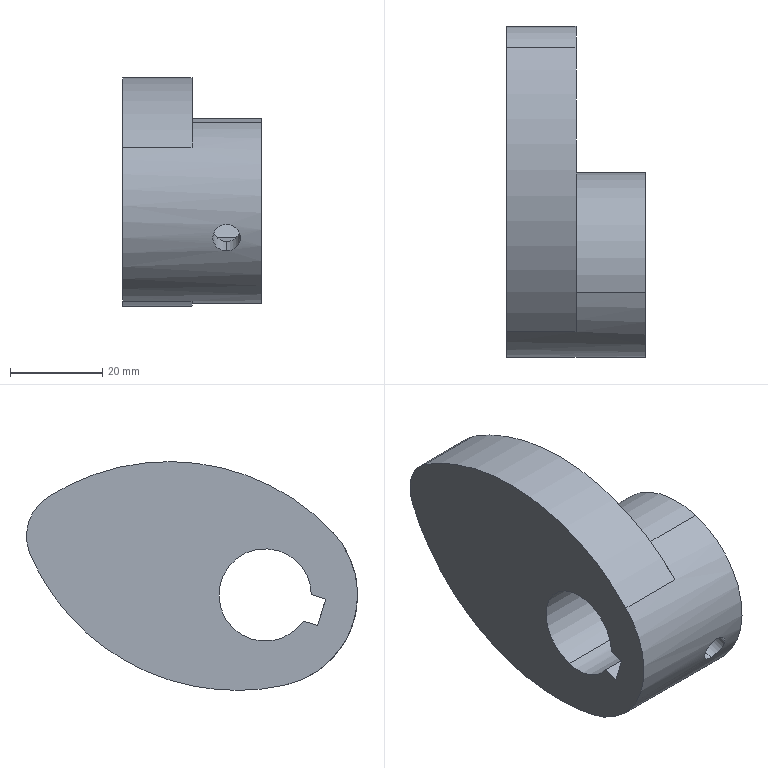Component | SolidWorks | ZL-11-11Cam2-1 | 1 solid | 20 faces | box 30 x 71.7 x 49.54 mm | volume 48547 mm3 | cylinder 13 | plane 7 | commonest cylinder face diameters 6 x4 20 x4 97.465 x3 40 x2
STEP:
#1=COLOUR_RGB('',0.7922,0.8196,0.9333);
#2=FILL_AREA_STYLE_COLOUR('',#1);
#3=FILL_AREA_STYLE('',(#2));
#4=SURFACE_STYLE_FILL_AREA(#3);
#5=SURFACE_SIDE_STYLE('',(#4));
#6=SURFACE_STYLE_USAGE(.BOTH.,#5);
#7=PRESENTATION_STYLE_ASSIGNMENT((#6));
#8=CARTESIAN_POINT('',(-2.2,4.601,-0.3247));
#9=VERTEX_POINT('',#8);
#10=CARTESIAN_POINT('',(-2.082,4.494,-0.3765));
#11=VERTEX_POINT('',#10);
#12=CARTESIAN_POINT('',(-2.2,4.601,-0.3247));
#13=CARTESIAN_POINT('',(-2.192,4.601,-0.3247));
#14=CARTESIAN_POINT('',(-2.184,4.601,-0.3251));
#15=CARTESIAN_POINT('',(-2.169,4.598,-0.3269));
#16=CARTESIAN_POINT('',(-2.161,4.596,-0.3282));
#17=CARTESIAN_POINT('',(-2.147,4.591,-0.3316));
#18=CARTESIAN_POINT('',(-2.14,4.588,-0.3337));
#19=CARTESIAN_POINT('',(-2.128,4.58,-0.3383));
#20=CARTESIAN_POINT('',(-2.122,4.576,-0.3408));
#21=CARTESIAN_POINT('',(-2.111,4.566,-0.3463));
#22=CARTESIAN_POINT('',(-2.106,4.561,-0.3491));
#23=CARTESIAN_POINT('',(-2.097,4.549,-0.3549));
#24=CARTESIAN_POINT('',(-2.094,4.543,-0.3579));
#25=CARTESIAN_POINT('',(-2.088,4.53,-0.3637));
#26=CARTESIAN_POINT('',(-2.085,4.523,-0.3664));
#27=CARTESIAN_POINT('',(-2.082,4.509,-0.3717));
#28=CARTESIAN_POINT('',(-2.082,4.501,-0.3742));
#29=CARTESIAN_POINT('',(-2.082,4.494,-0.3765));
#30=B_SPLINE_CURVE_WITH_KNOTS('',3,(#12,#13,#14,#15,#16,#17,#18,#19,#20,#21,#22,#23,#24,#25,#26,#27,#28,#29),.UNSPECIFIED.,.F.,.F.,(4,2,2,2,2,2,2,2,4),(0.009434,0.01002,0.01061,0.0112,0.01179,0.01238,0.01297,0.01356,0.01415),.UNSPECIFIED.);
#31=EDGE_CURVE('',#9,#11,#30,.T.);
#32=ORIENTED_EDGE('',*,*,#31,.F.);
#33=CARTESIAN_POINT('',(-2.2,4.719,-0.71));
#34=VERTEX_POINT('',#33);
#35=CARTESIAN_POINT('',(-2.2,4.722,-0.7185));
#36=DIRECTION('',(-0.,0.2922,-0.9564));
#37=VECTOR('',#36,39.37);
#38=LINE('',#35,#37);
#39=EDGE_CURVE('',#9,#34,#38,.T.);
#40=ORIENTED_EDGE('',*,*,#39,.T.);
#41=CARTESIAN_POINT('',(-2.082,4.609,-0.753));
#42=VERTEX_POINT('',#41);
#43=CARTESIAN_POINT('',(-2.082,4.609,-0.753));
#44=CARTESIAN_POINT('',(-2.082,4.616,-0.7508));
#45=CARTESIAN_POINT('',(-2.082,4.623,-0.7484));
#46=CARTESIAN_POINT('',(-2.085,4.638,-0.7435));
#47=CARTESIAN_POINT('',(-2.088,4.645,-0.7411));
#48=CARTESIAN_POINT('',(-2.094,4.658,-0.7361));
#49=CARTESIAN_POINT('',(-2.097,4.665,-0.7336));
#50=CARTESIAN_POINT('',(-2.106,4.677,-0.7288));
#51=CARTESIAN_POINT('',(-2.111,4.682,-0.7265));
#52=CARTESIAN_POINT('',(-2.122,4.692,-0.7223));
#53=CARTESIAN_POINT('',(-2.128,4.697,-0.7202));
#54=CARTESIAN_POINT('',(-2.14,4.705,-0.7167));
#55=CARTESIAN_POINT('',(-2.147,4.708,-0.7152));
#56=CARTESIAN_POINT('',(-2.162,4.714,-0.7126));
#57=CARTESIAN_POINT('',(-2.169,4.716,-0.7117));
#58=CARTESIAN_POINT('',(-2.184,4.718,-0.7103));
#59=CARTESIAN_POINT('',(-2.192,4.719,-0.71));
#60=CARTESIAN_POINT('',(-2.2,4.719,-0.71));
#61=B_SPLINE_CURVE_WITH_KNOTS('',3,(#43,#44,#45,#46,#47,#48,#49,#50,#51,#52,#53,#54,#55,#56,#57,#58,#59,#60),.UNSPECIFIED.,.F.,.F.,(4,2,2,2,2,2,2,2,4),(0.009393,0.00998,0.01057,0.01115,0.01174,0.01233,0.01292,0.0135,0.01409),.UNSPECIFIED.);
#62=EDGE_CURVE('',#42,#34,#61,.T.);
#63=ORIENTED_EDGE('',*,*,#62,.F.);
#64=CARTESIAN_POINT('',(-2.2,4.493,-0.779));
#65=VERTEX_POINT('',#64);
#66=CARTESIAN_POINT('',(-2.2,4.493,-0.779));
#67=CARTESIAN_POINT('',(-2.192,4.493,-0.779));
#68=CARTESIAN_POINT('',(-2.184,4.494,-0.7789));
#69=CARTESIAN_POINT('',(-2.169,4.497,-0.7785));
#70=CARTESIAN_POINT('',(-2.162,4.499,-0.7781));
#71=CARTESIAN_POINT('',(-2.147,4.505,-0.7772));
#72=CARTESIAN_POINT('',(-2.14,4.509,-0.7766));
#73=CARTESIAN_POINT('',(-2.128,4.517,-0.7751));
#74=CARTESIAN_POINT('',(-2.122,4.522,-0.7742));
#75=CARTESIAN_POINT('',(-2.111,4.533,-0.7721));
#76=CARTESIAN_POINT('',(-2.106,4.539,-0.771));
#77=CARTESIAN_POINT('',(-2.097,4.551,-0.7682));
#78=CARTESIAN_POINT('',(-2.094,4.558,-0.7667));
#79=CARTESIAN_POINT('',(-2.088,4.572,-0.7633));
#80=CARTESIAN_POINT('',(-2.085,4.579,-0.7615));
#81=CARTESIAN_POINT('',(-2.082,4.594,-0.7575));
#82=CARTESIAN_POINT('',(-2.082,4.601,-0.7553));
#83=CARTESIAN_POINT('',(-2.082,4.609,-0.753));
#84=B_SPLINE_CURVE_WITH_KNOTS('',3,(#66,#67,#68,#69,#70,#71,#72,#73,#74,#75,#76,#77,#78,#79,#80,#81,#82,#83),.UNSPECIFIED.,.F.,.F.,(4,2,2,2,2,2,2,2,4),(0.004697,0.005284,0.005871,0.006458,0.007045,0.007632,0.008219,0.008806,0.009393),.UNSPECIFIED.);
#85=EDGE_CURVE('',#65,#42,#84,.T.);
#86=ORIENTED_EDGE('',*,*,#85,.F.);
#87=CARTESIAN_POINT('',(-2.2,4.376,-0.3937));
#88=VERTEX_POINT('',#87);
#89=CARTESIAN_POINT('',(-2.2,4.496,-0.7876));
#90=DIRECTION('',(-0.,0.2922,-0.9564));
#91=VECTOR('',#90,39.37);
#92=LINE('',#89,#91);
#93=EDGE_CURVE('',#88,#65,#92,.T.);
#94=ORIENTED_EDGE('',*,*,#93,.F.);
#95=CARTESIAN_POINT('',(-2.082,4.494,-0.3765));
#96=CARTESIAN_POINT('',(-2.082,4.486,-0.3788));
#97=CARTESIAN_POINT('',(-2.082,4.479,-0.3808));
#98=CARTESIAN_POINT('',(-2.085,4.464,-0.3844));
#99=CARTESIAN_POINT('',(-2.088,4.457,-0.386));
#100=CARTESIAN_POINT('',(-2.097,4.436,-0.3898));
#101=CARTESIAN_POINT('',(-2.105,4.422,-0.3914));
#102=CARTESIAN_POINT('',(-2.122,4.406,-0.3928));
#103=CARTESIAN_POINT('',(-2.128,4.401,-0.3931));
#104=CARTESIAN_POINT('',(-2.14,4.392,-0.3935));
#105=CARTESIAN_POINT('',(-2.147,4.388,-0.3936));
#106=CARTESIAN_POINT('',(-2.161,4.382,-0.3937));
#107=CARTESIAN_POINT('',(-2.169,4.379,-0.3937));
#108=CARTESIAN_POINT('',(-2.184,4.376,-0.3937));
#109=CARTESIAN_POINT('',(-2.192,4.376,-0.3937));
#110=CARTESIAN_POINT('',(-2.2,4.376,-0.3937));
#111=B_SPLINE_CURVE_WITH_KNOTS('',3,(#95,#96,#97,#98,#99,#100,#101,#102,#103,#104,#105,#106,#107,#108,#109,#110),.UNSPECIFIED.,.F.,.F.,(4,2,2,2,2,2,2,4),(0.01415,0.01474,0.01533,0.01651,0.0171,0.01769,0.01828,0.01887),.UNSPECIFIED.);
#112=EDGE_CURVE('',#11,#88,#111,.T.);
#113=ORIENTED_EDGE('',*,*,#112,.F.);
#114=EDGE_LOOP('',(#32,#40,#63,#86,#94,#113));
#115=FACE_OUTER_BOUND('',#114,.T.);
#116=CARTESIAN_POINT('',(-2.2,4.609,-0.753));
#117=DIRECTION('',(-0.,0.2922,-0.9564));
#118=DIRECTION('',(0.,-0.9564,-0.2922));
#119=AXIS2_PLACEMENT_3D('',#116,#117,#118);
#120=CYLINDRICAL_SURFACE('',#119,0.1181);
#121=ADVANCED_FACE('',(#115),#120,.F.);
#122=CARTESIAN_POINT('',(-2.2,3.931,-0.2602));
#123=VERTEX_POINT('',#122);
#124=CARTESIAN_POINT('',(-2.2,3.862,-0.03428));
#125=VERTEX_POINT('',#124);
#126=CARTESIAN_POINT('',(-2.2,3.897,-0.1472));
#127=DIRECTION('',(0.,-0.9564,-0.2922));
#128=DIRECTION('',(0.,-0.2922,0.9564));
#129=AXIS2_PLACEMENT_3D('',#126,#127,#128);
#130=CIRCLE('',#129,0.1181);
#131=EDGE_CURVE('',#123,#125,#130,.T.);
#132=ORIENTED_EDGE('',*,*,#131,.F.);
#133=CARTESIAN_POINT('',(-2.2,3.669,-0.3404));
#134=VERTEX_POINT('',#133);
#135=CARTESIAN_POINT('',(-2.2,3.66,-0.343));
#136=DIRECTION('',(0.,-0.9564,-0.2922));
#137=VECTOR('',#136,39.37);
#138=LINE('',#135,#137);
#139=EDGE_CURVE('',#123,#134,#138,.T.);
#140=ORIENTED_EDGE('',*,*,#139,.T.);
#141=CARTESIAN_POINT('',(-2.2,3.6,-0.1145));
#142=VERTEX_POINT('',#141);
#143=CARTESIAN_POINT('',(-2.2,3.6,-0.1145));
#144=CARTESIAN_POINT('',(-2.192,3.6,-0.1145));
#145=CARTESIAN_POINT('',(-2.184,3.6,-0.1153));
#146=CARTESIAN_POINT('',(-2.169,3.6,-0.1183));
#147=CARTESIAN_POINT('',(-2.162,3.601,-0.1206));
#148=CARTESIAN_POINT('',(-2.147,3.602,-0.1265));
#149=CARTESIAN_POINT('',(-2.141,3.602,-0.1301));
#150=CARTESIAN_POINT('',(-2.128,3.604,-0.1386));
#151=CARTESIAN_POINT('',(-2.122,3.604,-0.1435));
#152=CARTESIAN_POINT('',(-2.111,3.607,-0.1543));
#153=CARTESIAN_POINT('',(-2.106,3.608,-0.1601));
#154=CARTESIAN_POINT('',(-2.097,3.61,-0.1728));
#155=CARTESIAN_POINT('',(-2.094,3.612,-0.1795));
#156=CARTESIAN_POINT('',(-2.088,3.615,-0.1933));
#157=CARTESIAN_POINT('',(-2.085,3.617,-0.2006));
#158=CARTESIAN_POINT('',(-2.082,3.621,-0.2153));
#159=CARTESIAN_POINT('',(-2.082,3.623,-0.2226));
#160=CARTESIAN_POINT('',(-2.082,3.628,-0.2374));
#161=CARTESIAN_POINT('',(-2.082,3.63,-0.2449));
#162=CARTESIAN_POINT('',(-2.085,3.635,-0.2592));
#163=CARTESIAN_POINT('',(-2.088,3.638,-0.2662));
#164=CARTESIAN_POINT('',(-2.094,3.643,-0.2796));
#165=CARTESIAN_POINT('',(-2.097,3.645,-0.2861));
#166=CARTESIAN_POINT('',(-2.106,3.65,-0.298));
#167=CARTESIAN_POINT('',(-2.111,3.652,-0.3035));
#168=CARTESIAN_POINT('',(-2.122,3.657,-0.3137));
#169=CARTESIAN_POINT('',(-2.128,3.658,-0.3182));
#170=CARTESIAN_POINT('',(-2.14,3.662,-0.3261));
#171=CARTESIAN_POINT('',(-2.147,3.664,-0.3295));
#172=CARTESIAN_POINT('',(-2.162,3.666,-0.3349));
#173=CARTESIAN_POINT('',(-2.169,3.667,-0.337));
#174=CARTESIAN_POINT('',(-2.184,3.668,-0.3397));
#175=CARTESIAN_POINT('',(-2.192,3.669,-0.3404));
#176=CARTESIAN_POINT('',(-2.2,3.669,-0.3404));
#177=B_SPLINE_CURVE_WITH_KNOTS('',3,(#143,#144,#145,#146,#147,#148,#149,#150,#151,#152,#153,#154,#155,#156,#157,#158,#159,#160,#161,#162,#163,#164,#165,#166,#167,#168,#169,#170,#171,#172,#173,#174,#175,#176),.UNSPECIFIED.,.F.,.F.,(4,2,2,2,2,2,2,2,2,2,2,2,2,2,2,2,4),(0.,0.000587,0.001174,0.001761,0.002348,0.002935,0.003522,0.004109,0.004696,0.005283,0.00587,0.006457,0.007044,0.007631,0.008219,0.008806,0.009393),.UNSPECIFIED.);
#178=EDGE_CURVE('',#142,#134,#177,.T.);
#179=ORIENTED_EDGE('',*,*,#178,.F.);
#180=CARTESIAN_POINT('',(-2.2,3.591,-0.1171));
#181=DIRECTION('',(0.,-0.9564,-0.2922));
#182=VECTOR('',#181,39.37);
#183=LINE('',#180,#182);
#184=EDGE_CURVE('',#125,#142,#183,.T.);
#185=ORIENTED_EDGE('',*,*,#184,.F.);
#186=EDGE_LOOP('',(#132,#140,#179,#185));
#187=FACE_OUTER_BOUND('',#186,.T.);
#188=CARTESIAN_POINT('',(-2.2,3.626,-0.2301));
#189=DIRECTION('',(0.,-0.9564,-0.2922));
#190=DIRECTION('',(0.,-0.2922,0.9564));
#191=AXIS2_PLACEMENT_3D('',#188,#189,#190);
#192=CYLINDRICAL_SURFACE('',#191,0.1181);
#193=ADVANCED_FACE('',(#187),#192,.F.);
#194=CARTESIAN_POINT('',(-3.086,4.264,0.3765));
#195=VERTEX_POINT('',#194);
#196=CARTESIAN_POINT('',(-3.086,3.985,0.003219));
#197=VERTEX_POINT('',#196);
#198=CARTESIAN_POINT('',(-3.086,4.379,0.));
#199=DIRECTION('',(1.,0.,-0.));
#200=DIRECTION('',(0.,0.2922,-0.9564));
#201=AXIS2_PLACEMENT_3D('',#198,#199,#200);
#202=CIRCLE('',#201,0.3937);
#203=EDGE_CURVE('',#195,#197,#202,.T.);
#204=ORIENTED_EDGE('',*,*,#203,.F.);
#205=CARTESIAN_POINT('',(-1.904,4.264,0.3765));
#206=VERTEX_POINT('',#205);
#207=CARTESIAN_POINT('',(-3.086,4.264,0.3765));
#208=DIRECTION('',(1.,0.,-0.));
#209=VECTOR('',#208,39.37);
#210=LINE('',#207,#209);
#211=EDGE_CURVE('',#195,#206,#210,.T.);
#212=ORIENTED_EDGE('',*,*,#211,.T.);
#213=CARTESIAN_POINT('',(-1.904,3.985,0.003219));
#214=VERTEX_POINT('',#213);
#215=CARTESIAN_POINT('',(-1.904,4.379,-0.));
#216=DIRECTION('',(1.,0.,-0.));
#217=DIRECTION('',(0.,0.2922,-0.9564));
#218=AXIS2_PLACEMENT_3D('',#215,#216,#217);
#219=CIRCLE('',#218,0.3937);
#220=EDGE_CURVE('',#206,#214,#219,.T.);
#221=ORIENTED_EDGE('',*,*,#220,.T.);
#222=CARTESIAN_POINT('',(-3.086,3.985,0.003219));
#223=DIRECTION('',(1.,0.,-0.));
#224=VECTOR('',#223,39.37);
#225=LINE('',#222,#224);
#226=EDGE_CURVE('',#197,#214,#225,.T.);
#227=ORIENTED_EDGE('',*,*,#226,.F.);
#228=EDGE_LOOP('',(#204,#212,#221,#227));
#229=FACE_OUTER_BOUND('',#228,.T.);
#230=CARTESIAN_POINT('',(-3.086,4.379,0.));
#231=DIRECTION('',(1.,0.,-0.));
#232=DIRECTION('',(0.,0.2922,-0.9564));
#233=AXIS2_PLACEMENT_3D('',#230,#231,#232);
#234=CYLINDRICAL_SURFACE('',#233,0.3937);
#235=ADVANCED_FACE('',(#229),#234,.F.);
#236=ORIENTED_EDGE('',*,*,#211,.F.);
#237=CARTESIAN_POINT('',(-3.086,4.494,-0.3765));
#238=VERTEX_POINT('',#237);
#239=CARTESIAN_POINT('',(-3.086,4.379,0.));
#240=DIRECTION('',(1.,0.,-0.));
#241=DIRECTION('',(0.,0.2922,-0.9564));
#242=AXIS2_PLACEMENT_3D('',#239,#240,#241);
#243=CIRCLE('',#242,0.3937);
#244=EDGE_CURVE('',#238,#195,#243,.T.);
#245=ORIENTED_EDGE('',*,*,#244,.F.);
#246=CARTESIAN_POINT('',(-2.318,4.494,-0.3765));
#247=VERTEX_POINT('',#246);
#248=CARTESIAN_POINT('',(-3.086,4.494,-0.3765));
#249=DIRECTION('',(1.,0.,-0.));
#250=VECTOR('',#249,39.37);
#251=LINE('',#248,#250);
#252=EDGE_CURVE('',#238,#247,#251,.T.);
#253=ORIENTED_EDGE('',*,*,#252,.T.);
#254=CARTESIAN_POINT('',(-2.318,4.494,-0.3765));
#255=CARTESIAN_POINT('',(-2.318,4.501,-0.3743));
#256=CARTESIAN_POINT('',(-2.317,4.509,-0.3717));
#257=CARTESIAN_POINT('',(-2.314,4.523,-0.3664));
#258=CARTESIAN_POINT('',(-2.312,4.53,-0.3636));
#259=CARTESIAN_POINT('',(-2.306,4.543,-0.3579));
#260=CARTESIAN_POINT('',(-2.302,4.549,-0.3549));
#261=CARTESIAN_POINT('',(-2.294,4.561,-0.3491));
#262=CARTESIAN_POINT('',(-2.289,4.566,-0.3462));
#263=CARTESIAN_POINT('',(-2.278,4.576,-0.3408));
#264=CARTESIAN_POINT('',(-2.272,4.58,-0.3383));
#265=CARTESIAN_POINT('',(-2.259,4.588,-0.3337));
#266=CARTESIAN_POINT('',(-2.252,4.591,-0.3316));
#267=CARTESIAN_POINT('',(-2.238,4.596,-0.3282));
#268=CARTESIAN_POINT('',(-2.231,4.598,-0.3269));
#269=CARTESIAN_POINT('',(-2.215,4.601,-0.3251));
#270=CARTESIAN_POINT('',(-2.207,4.601,-0.3247));
#271=CARTESIAN_POINT('',(-2.2,4.601,-0.3247));
#272=B_SPLINE_CURVE_WITH_KNOTS('',3,(#254,#255,#256,#257,#258,#259,#260,#261,#262,#263,#264,#265,#266,#267,#268,#269,#270,#271),.UNSPECIFIED.,.F.,.F.,(4,2,2,2,2,2,2,2,4),(0.004718,0.005308,0.005897,0.006487,0.007076,0.007665,0.008255,0.008844,0.009434),.UNSPECIFIED.);
#273=EDGE_CURVE('',#247,#9,#272,.T.);
#274=ORIENTED_EDGE('',*,*,#273,.T.);
#275=ORIENTED_EDGE('',*,*,#31,.T.);
#276=CARTESIAN_POINT('',(-1.904,4.494,-0.3765));
#277=VERTEX_POINT('',#276);
#278=CARTESIAN_POINT('',(-3.086,4.494,-0.3765));
#279=DIRECTION('',(1.,0.,-0.));
#280=VECTOR('',#279,39.37);
#281=LINE('',#278,#280);
#282=EDGE_CURVE('',#11,#277,#281,.T.);
#283=ORIENTED_EDGE('',*,*,#282,.T.);
#284=CARTESIAN_POINT('',(-1.904,4.379,-0.));
#285=DIRECTION('',(1.,0.,-0.));
#286=DIRECTION('',(0.,0.2922,-0.9564));
#287=AXIS2_PLACEMENT_3D('',#284,#285,#286);
#288=CIRCLE('',#287,0.3937);
#289=EDGE_CURVE('',#277,#206,#288,.T.);
#290=ORIENTED_EDGE('',*,*,#289,.T.);
#291=EDGE_LOOP('',(#236,#245,#253,#274,#275,#283,#290));
#292=FACE_OUTER_BOUND('',#291,.T.);
#293=CARTESIAN_POINT('',(-3.086,4.379,0.));
#294=DIRECTION('',(1.,0.,-0.));
#295=DIRECTION('',(0.,0.2922,-0.9564));
#296=AXIS2_PLACEMENT_3D('',#293,#294,#295);
#297=CYLINDRICAL_SURFACE('',#296,0.3937);
#298=ADVANCED_FACE('',(#292),#297,.F.);
#299=CARTESIAN_POINT('',(-2.495,4.609,-0.753));
#300=VERTEX_POINT('',#299);
#301=CARTESIAN_POINT('',(-2.495,4.149,0.753));
#302=VERTEX_POINT('',#301);
#303=CARTESIAN_POINT('',(-2.495,4.379,-0.));
#304=DIRECTION('',(1.,0.,-0.));
#305=DIRECTION('',(0.,0.2922,-0.9564));
#306=AXIS2_PLACEMENT_3D('',#303,#304,#305);
#307=CIRCLE('',#306,0.7874);
#308=EDGE_CURVE('',#300,#302,#307,.T.);
#309=ORIENTED_EDGE('',*,*,#308,.T.);
#310=CARTESIAN_POINT('',(-1.904,4.149,0.753));
#311=VERTEX_POINT('',#310);
#312=CARTESIAN_POINT('',(-3.086,4.149,0.753));
#313=DIRECTION('',(1.,0.,-0.));
#314=VECTOR('',#313,39.37);
#315=LINE('',#312,#314);
#316=EDGE_CURVE('',#302,#311,#315,.T.);
#317=ORIENTED_EDGE('',*,*,#316,.T.);
#318=CARTESIAN_POINT('',(-1.904,4.609,-0.753));
#319=VERTEX_POINT('',#318);
#320=CARTESIAN_POINT('',(-1.904,4.379,-0.));
#321=DIRECTION('',(1.,0.,-0.));
#322=DIRECTION('',(-0.,0.2922,-0.9564));
#323=AXIS2_PLACEMENT_3D('',#320,#321,#322);
#324=CIRCLE('',#323,0.7874);
#325=EDGE_CURVE('',#319,#311,#324,.T.);
#326=ORIENTED_EDGE('',*,*,#325,.F.);
#327=CARTESIAN_POINT('',(-3.086,4.609,-0.753));
#328=DIRECTION('',(1.,0.,-0.));
#329=VECTOR('',#328,39.37);
#330=LINE('',#327,#329);
#331=EDGE_CURVE('',#42,#319,#330,.T.);
#332=ORIENTED_EDGE('',*,*,#331,.F.);
#333=ORIENTED_EDGE('',*,*,#62,.T.);
#334=CARTESIAN_POINT('',(-2.318,4.609,-0.753));
#335=VERTEX_POINT('',#334);
#336=CARTESIAN_POINT('',(-2.2,4.719,-0.71));
#337=CARTESIAN_POINT('',(-2.208,4.719,-0.71));
#338=CARTESIAN_POINT('',(-2.215,4.718,-0.7103));
#339=CARTESIAN_POINT('',(-2.23,4.716,-0.7116));
#340=CARTESIAN_POINT('',(-2.238,4.714,-0.7126));
#341=CARTESIAN_POINT('',(-2.252,4.708,-0.7152));
#342=CARTESIAN_POINT('',(-2.259,4.705,-0.7167));
#343=CARTESIAN_POINT('',(-2.272,4.697,-0.7202));
#344=CARTESIAN_POINT('',(-2.278,4.692,-0.7222));
#345=CARTESIAN_POINT('',(-2.289,4.682,-0.7265));
#346=CARTESIAN_POINT('',(-2.294,4.677,-0.7288));
#347=CARTESIAN_POINT('',(-2.302,4.665,-0.7336));
#348=CARTESIAN_POINT('',(-2.306,4.658,-0.7361));
#349=CARTESIAN_POINT('',(-2.312,4.645,-0.741));
#350=CARTESIAN_POINT('',(-2.314,4.638,-0.7435));
#351=CARTESIAN_POINT('',(-2.317,4.624,-0.7484));
#352=CARTESIAN_POINT('',(-2.318,4.616,-0.7508));
#353=CARTESIAN_POINT('',(-2.318,4.609,-0.753));
#354=B_SPLINE_CURVE_WITH_KNOTS('',3,(#336,#337,#338,#339,#340,#341,#342,#343,#344,#345,#346,#347,#348,#349,#350,#351,#352,#353),.UNSPECIFIED.,.F.,.F.,(4,2,2,2,2,2,2,2,4),(0.01409,0.01468,0.01526,0.01585,0.01644,0.01702,0.01761,0.0182,0.01878),.UNSPECIFIED.);
#355=EDGE_CURVE('',#34,#335,#354,.T.);
#356=ORIENTED_EDGE('',*,*,#355,.T.);
#357=CARTESIAN_POINT('',(-3.086,4.609,-0.753));
#358=DIRECTION('',(1.,0.,-0.));
#359=VECTOR('',#358,39.37);
#360=LINE('',#357,#359);
#361=EDGE_CURVE('',#300,#335,#360,.T.);
#362=ORIENTED_EDGE('',*,*,#361,.F.);
#363=EDGE_LOOP('',(#309,#317,#326,#332,#333,#356,#362));
#364=FACE_OUTER_BOUND('',#363,.T.);
#365=CARTESIAN_POINT('',(-3.086,4.379,0.));
#366=DIRECTION('',(1.,0.,-0.));
#367=DIRECTION('',(0.,0.2922,-0.9564));
#368=AXIS2_PLACEMENT_3D('',#365,#366,#367);
#369=CYLINDRICAL_SURFACE('',#368,0.7874);
#370=ADVANCED_FACE('',(#364),#369,.T.);
#371=CARTESIAN_POINT('',(-3.086,5.181,-0.7297));
#372=VERTEX_POINT('',#371);
#373=CARTESIAN_POINT('',(-3.086,4.211,-0.7693));
#374=VERTEX_POINT('',#373);
#375=CARTESIAN_POINT('',(-3.086,4.62,1.105));
#376=DIRECTION('',(-1.,-0.,0.));
#377=DIRECTION('',(0.,-0.2922,0.9564));
#378=AXIS2_PLACEMENT_3D('',#375,#376,#377);
#379=CIRCLE('',#378,1.919);
#380=EDGE_CURVE('',#372,#374,#379,.T.);
#381=ORIENTED_EDGE('',*,*,#380,.F.);
#382=CARTESIAN_POINT('',(-2.495,5.181,-0.7297));
#383=VERTEX_POINT('',#382);
#384=CARTESIAN_POINT('',(-3.086,5.181,-0.7297));
#385=DIRECTION('',(1.,0.,-0.));
#386=VECTOR('',#385,39.37);
#387=LINE('',#384,#386);
#388=EDGE_CURVE('',#372,#383,#387,.T.);
#389=ORIENTED_EDGE('',*,*,#388,.T.);
#390=CARTESIAN_POINT('',(-2.495,4.211,-0.7693));
#391=VERTEX_POINT('',#390);
#392=CARTESIAN_POINT('',(-2.495,4.62,1.105));
#393=DIRECTION('',(-1.,-0.,0.));
#394=DIRECTION('',(0.,-0.2922,0.9564));
#395=AXIS2_PLACEMENT_3D('',#392,#393,#394);
#396=CIRCLE('',#395,1.919);
#397=EDGE_CURVE('',#383,#391,#396,.T.);
#398=ORIENTED_EDGE('',*,*,#397,.T.);
#399=CARTESIAN_POINT('',(-3.086,4.211,-0.7693));
#400=DIRECTION('',(1.,0.,-0.));
#401=VECTOR('',#400,39.37);
#402=LINE('',#399,#401);
#403=EDGE_CURVE('',#374,#391,#402,.T.);
#404=ORIENTED_EDGE('',*,*,#403,.F.);
#405=EDGE_LOOP('',(#381,#389,#398,#404));
#406=FACE_OUTER_BOUND('',#405,.T.);
#407=CARTESIAN_POINT('',(-3.086,4.62,1.105));
#408=DIRECTION('',(1.,0.,-0.));
#409=DIRECTION('',(-0.,0.2922,-0.9564));
#410=AXIS2_PLACEMENT_3D('',#407,#408,#409);
#411=CYLINDRICAL_SURFACE('',#410,1.919);
#412=ADVANCED_FACE('',(#406),#411,.T.);
#413=CARTESIAN_POINT('',(-3.086,3.862,-0.03429));
#414=VERTEX_POINT('',#413);
#415=CARTESIAN_POINT('',(-3.086,3.862,-0.03429));
#416=DIRECTION('',(1.,0.,-0.));
#417=VECTOR('',#416,39.37);
#418=LINE('',#415,#417);
#419=EDGE_CURVE('',#414,#125,#418,.T.);
#420=ORIENTED_EDGE('',*,*,#419,.T.);
#421=CARTESIAN_POINT('',(-2.2,3.897,-0.1472));
#422=DIRECTION('',(0.,-0.9564,-0.2922));
#423=DIRECTION('',(0.,-0.2922,0.9564));
#424=AXIS2_PLACEMENT_3D('',#421,#422,#423);
#425=CIRCLE('',#424,0.1181);
#426=EDGE_CURVE('',#125,#123,#425,.T.);
#427=ORIENTED_EDGE('',*,*,#426,.T.);
#428=CARTESIAN_POINT('',(-3.086,3.931,-0.2602));
#429=VERTEX_POINT('',#428);
#430=CARTESIAN_POINT('',(-3.086,3.931,-0.2602));
#431=DIRECTION('',(1.,0.,-0.));
#432=VECTOR('',#431,39.37);
#433=LINE('',#430,#432);
#434=EDGE_CURVE('',#429,#123,#433,.T.);
#435=ORIENTED_EDGE('',*,*,#434,.F.);
#436=CARTESIAN_POINT('',(-3.086,3.753,0.3245));
#437=DIRECTION('',(0.,-0.2922,0.9564));
#438=VECTOR('',#437,39.37);
#439=LINE('',#436,#438);
#440=EDGE_CURVE('',#429,#414,#439,.T.);
#441=ORIENTED_EDGE('',*,*,#440,.T.);
#442=EDGE_LOOP('',(#420,#427,#435,#441));
#443=FACE_OUTER_BOUND('',#442,.T.);
#444=CARTESIAN_POINT('',(-3.086,3.862,-0.03429));
#445=DIRECTION('',(0.,-0.9564,-0.2922));
#446=DIRECTION('',(0.,-0.2922,0.9564));
#447=AXIS2_PLACEMENT_3D('',#444,#445,#446);
#448=PLANE('',#447);
#449=ADVANCED_FACE('',(#443),#448,.F.);
#450=CARTESIAN_POINT('',(-2.495,4.379,-0.));
#451=DIRECTION('',(1.,0.,-0.));
#452=DIRECTION('',(0.,0.2922,-0.9564));
#453=AXIS2_PLACEMENT_3D('',#450,#451,#452);
#454=CIRCLE('',#453,0.7874);
#455=EDGE_CURVE('',#391,#300,#454,.T.);
#456=ORIENTED_EDGE('',*,*,#455,.F.);
#457=ORIENTED_EDGE('',*,*,#397,.F.);
#458=CARTESIAN_POINT('',(-2.495,6.382,0.3457));
#459=VERTEX_POINT('',#458);
#460=CARTESIAN_POINT('',(-2.495,4.62,1.105));
#461=DIRECTION('',(-1.,-0.,0.));
#462=DIRECTION('',(0.,-0.2922,0.9564));
#463=AXIS2_PLACEMENT_3D('',#460,#461,#462);
#464=CIRCLE('',#463,1.919);
#465=EDGE_CURVE('',#459,#383,#464,.T.);
#466=ORIENTED_EDGE('',*,*,#465,.F.);
#467=CARTESIAN_POINT('',(-2.495,6.233,0.8328));
#468=VERTEX_POINT('',#467);
#469=CARTESIAN_POINT('',(-2.495,6.02,0.5016));
#470=DIRECTION('',(-1.,-0.,0.));
#471=DIRECTION('',(0.,-0.2922,0.9564));
#472=AXIS2_PLACEMENT_3D('',#469,#470,#471);
#473=CIRCLE('',#472,0.3937);
#474=EDGE_CURVE('',#468,#459,#473,.T.);
#475=ORIENTED_EDGE('',*,*,#474,.F.);
#476=CARTESIAN_POINT('',(-2.495,3.81,0.5441));
#477=VERTEX_POINT('',#476);
#478=CARTESIAN_POINT('',(-2.495,5.196,-0.7816));
#479=DIRECTION('',(-1.,-0.,0.));
#480=DIRECTION('',(-0.,0.2922,-0.9564));
#481=AXIS2_PLACEMENT_3D('',#478,#479,#480);
#482=CIRCLE('',#481,1.919);
#483=EDGE_CURVE('',#477,#468,#482,.T.);
#484=ORIENTED_EDGE('',*,*,#483,.F.);
#485=CARTESIAN_POINT('',(-2.495,4.379,-0.));
#486=DIRECTION('',(1.,0.,-0.));
#487=DIRECTION('',(0.,0.2922,-0.9564));
#488=AXIS2_PLACEMENT_3D('',#485,#486,#487);
#489=CIRCLE('',#488,0.7874);
#490=EDGE_CURVE('',#302,#477,#489,.T.);
#491=ORIENTED_EDGE('',*,*,#490,.F.);
#492=ORIENTED_EDGE('',*,*,#308,.F.);
#493=EDGE_LOOP('',(#456,#457,#466,#475,#484,#491,#492));
#494=FACE_OUTER_BOUND('',#493,.T.);
#495=CARTESIAN_POINT('',(-2.495,5.32,0.8034));
#496=DIRECTION('',(-1.,-0.,0.));
#497=DIRECTION('',(0.,-0.2922,0.9564));
#498=AXIS2_PLACEMENT_3D('',#495,#496,#497);
#499=PLANE('',#498);
#500=ADVANCED_FACE('',(#494),#499,.F.);
#501=ORIENTED_EDGE('',*,*,#474,.T.);
#502=CARTESIAN_POINT('',(-3.086,6.382,0.3457));
#503=VERTEX_POINT('',#502);
#504=CARTESIAN_POINT('',(-3.086,6.382,0.3457));
#505=DIRECTION('',(1.,0.,-0.));
#506=VECTOR('',#505,39.37);
#507=LINE('',#504,#506);
#508=EDGE_CURVE('',#503,#459,#507,.T.);
#509=ORIENTED_EDGE('',*,*,#508,.F.);
#510=CARTESIAN_POINT('',(-3.086,6.233,0.8328));
#511=VERTEX_POINT('',#510);
#512=CARTESIAN_POINT('',(-3.086,6.02,0.5016));
#513=DIRECTION('',(-1.,-0.,0.));
#514=DIRECTION('',(0.,-0.2922,0.9564));
#515=AXIS2_PLACEMENT_3D('',#512,#513,#514);
#516=CIRCLE('',#515,0.3937);
#517=EDGE_CURVE('',#511,#503,#516,.T.);
#518=ORIENTED_EDGE('',*,*,#517,.F.);
#519=CARTESIAN_POINT('',(-3.086,6.233,0.8328));
#520=DIRECTION('',(1.,0.,-0.));
#521=VECTOR('',#520,39.37);
#522=LINE('',#519,#521);
#523=EDGE_CURVE('',#511,#468,#522,.T.);
#524=ORIENTED_EDGE('',*,*,#523,.T.);
#525=EDGE_LOOP('',(#501,#509,#518,#524));
#526=FACE_OUTER_BOUND('',#525,.T.);
#527=CARTESIAN_POINT('',(-3.086,6.02,0.5016));
#528=DIRECTION('',(1.,0.,-0.));
#529=DIRECTION('',(0.,0.2922,-0.9564));
#530=AXIS2_PLACEMENT_3D('',#527,#528,#529);
#531=CYLINDRICAL_SURFACE('',#530,0.3937);
#532=ADVANCED_FACE('',(#526),#531,.T.);
#533=ORIENTED_EDGE('',*,*,#388,.F.);
#534=CARTESIAN_POINT('',(-3.086,4.62,1.105));
#535=DIRECTION('',(-1.,-0.,0.));
#536=DIRECTION('',(0.,-0.2922,0.9564));
#537=AXIS2_PLACEMENT_3D('',#534,#535,#536);
#538=CIRCLE('',#537,1.919);
#539=EDGE_CURVE('',#503,#372,#538,.T.);
#540=ORIENTED_EDGE('',*,*,#539,.F.);
#541=ORIENTED_EDGE('',*,*,#508,.T.);
#542=ORIENTED_EDGE('',*,*,#465,.T.);
#543=EDGE_LOOP('',(#533,#540,#541,#542));
#544=FACE_OUTER_BOUND('',#543,.T.);
#545=CARTESIAN_POINT('',(-3.086,4.62,1.105));
#546=DIRECTION('',(1.,0.,-0.));
#547=DIRECTION('',(-0.,0.2922,-0.9564));
#548=AXIS2_PLACEMENT_3D('',#545,#546,#547);
#549=CYLINDRICAL_SURFACE('',#548,1.919);
#550=ADVANCED_FACE('',(#544),#549,.T.);
#551=ORIENTED_EDGE('',*,*,#316,.F.);
#552=ORIENTED_EDGE('',*,*,#490,.T.);
#553=CARTESIAN_POINT('',(-3.086,3.81,0.5441));
#554=VERTEX_POINT('',#553);
#555=CARTESIAN_POINT('',(-3.086,3.81,0.5441));
#556=DIRECTION('',(1.,0.,-0.));
#557=VECTOR('',#556,39.37);
#558=LINE('',#555,#557);
#559=EDGE_CURVE('',#554,#477,#558,.T.);
#560=ORIENTED_EDGE('',*,*,#559,.F.);
#561=CARTESIAN_POINT('',(-3.086,4.379,0.));
#562=DIRECTION('',(-1.,-0.,0.));
#563=DIRECTION('',(0.,-0.2922,0.9564));
#564=AXIS2_PLACEMENT_3D('',#561,#562,#563);
#565=CIRCLE('',#564,0.7874);
#566=EDGE_CURVE('',#374,#554,#565,.T.);
#567=ORIENTED_EDGE('',*,*,#566,.F.);
#568=ORIENTED_EDGE('',*,*,#403,.T.);
#569=ORIENTED_EDGE('',*,*,#455,.T.);
#570=ORIENTED_EDGE('',*,*,#361,.T.);
#571=CARTESIAN_POINT('',(-2.318,4.609,-0.753));
#572=CARTESIAN_POINT('',(-2.318,4.601,-0.7553));
#573=CARTESIAN_POINT('',(-2.317,4.594,-0.7575));
#574=CARTESIAN_POINT('',(-2.314,4.579,-0.7615));
#575=CARTESIAN_POINT('',(-2.312,4.572,-0.7633));
#576=CARTESIAN_POINT('',(-2.306,4.558,-0.7667));
#577=CARTESIAN_POINT('',(-2.302,4.552,-0.7682));
#578=CARTESIAN_POINT('',(-2.294,4.539,-0.771));
#579=CARTESIAN_POINT('',(-2.289,4.533,-0.7722));
#580=CARTESIAN_POINT('',(-2.278,4.522,-0.7742));
#581=CARTESIAN_POINT('',(-2.272,4.517,-0.7751));
#582=CARTESIAN_POINT('',(-2.259,4.509,-0.7766));
#583=CARTESIAN_POINT('',(-2.252,4.505,-0.7772));
#584=CARTESIAN_POINT('',(-2.238,4.499,-0.7781));
#585=CARTESIAN_POINT('',(-2.23,4.497,-0.7785));
#586=CARTESIAN_POINT('',(-2.215,4.494,-0.7789));
#587=CARTESIAN_POINT('',(-2.207,4.493,-0.779));
#588=CARTESIAN_POINT('',(-2.2,4.493,-0.779));
#589=B_SPLINE_CURVE_WITH_KNOTS('',3,(#571,#572,#573,#574,#575,#576,#577,#578,#579,#580,#581,#582,#583,#584,#585,#586,#587,#588),.UNSPECIFIED.,.F.,.F.,(4,2,2,2,2,2,2,2,4),(0.,0.0005872,0.001174,0.001762,0.002349,0.002936,0.003523,0.00411,0.004697),.UNSPECIFIED.);
#590=EDGE_CURVE('',#335,#65,#589,.T.);
#591=ORIENTED_EDGE('',*,*,#590,.T.);
#592=ORIENTED_EDGE('',*,*,#85,.T.);
#593=ORIENTED_EDGE('',*,*,#331,.T.);
#594=CARTESIAN_POINT('',(-1.904,4.379,-0.));
#595=DIRECTION('',(1.,0.,-0.));
#596=DIRECTION('',(-0.,0.2922,-0.9564));
#597=AXIS2_PLACEMENT_3D('',#594,#595,#596);
#598=CIRCLE('',#597,0.7874);
#599=EDGE_CURVE('',#311,#319,#598,.T.);
#600=ORIENTED_EDGE('',*,*,#599,.F.);
#601=EDGE_LOOP('',(#551,#552,#560,#567,#568,#569,#570,#591,#592,#593,#600));
#602=FACE_OUTER_BOUND('',#601,.T.);
#603=ORIENTED_EDGE('',*,*,#178,.T.);
#604=CARTESIAN_POINT('',(-2.2,3.669,-0.3404));
#605=CARTESIAN_POINT('',(-2.207,3.669,-0.3404));
#606=CARTESIAN_POINT('',(-2.215,3.668,-0.3397));
#607=CARTESIAN_POINT('',(-2.23,3.667,-0.337));
#608=CARTESIAN_POINT('',(-2.238,3.666,-0.3349));
#609=CARTESIAN_POINT('',(-2.252,3.664,-0.3295));
#610=CARTESIAN_POINT('',(-2.259,3.662,-0.3261));
#611=CARTESIAN_POINT('',(-2.272,3.658,-0.3182));
#612=CARTESIAN_POINT('',(-2.278,3.656,-0.3137));
#613=CARTESIAN_POINT('',(-2.289,3.652,-0.3037));
#614=CARTESIAN_POINT('',(-2.294,3.65,-0.298));
#615=CARTESIAN_POINT('',(-2.302,3.645,-0.2861));
#616=CARTESIAN_POINT('',(-2.306,3.643,-0.2798));
#617=CARTESIAN_POINT('',(-2.312,3.638,-0.2663));
#618=CARTESIAN_POINT('',(-2.314,3.635,-0.2592));
#619=CARTESIAN_POINT('',(-2.317,3.63,-0.2449));
#620=CARTESIAN_POINT('',(-2.318,3.628,-0.2376));
#621=CARTESIAN_POINT('',(-2.318,3.623,-0.2227));
#622=CARTESIAN_POINT('',(-2.317,3.621,-0.2153));
#623=CARTESIAN_POINT('',(-2.314,3.617,-0.2007));
#624=CARTESIAN_POINT('',(-2.312,3.615,-0.1934));
#625=CARTESIAN_POINT('',(-2.306,3.612,-0.1795));
#626=CARTESIAN_POINT('',(-2.302,3.611,-0.1729));
#627=CARTESIAN_POINT('',(-2.294,3.608,-0.1603));
#628=CARTESIAN_POINT('',(-2.289,3.607,-0.1543));
#629=CARTESIAN_POINT('',(-2.278,3.605,-0.1436));
#630=CARTESIAN_POINT('',(-2.272,3.604,-0.1387));
#631=CARTESIAN_POINT('',(-2.259,3.602,-0.1301));
#632=CARTESIAN_POINT('',(-2.252,3.602,-0.1265));
#633=CARTESIAN_POINT('',(-2.238,3.601,-0.1206));
#634=CARTESIAN_POINT('',(-2.23,3.6,-0.1183));
#635=CARTESIAN_POINT('',(-2.215,3.6,-0.1153));
#636=CARTESIAN_POINT('',(-2.208,3.6,-0.1145));
#637=CARTESIAN_POINT('',(-2.2,3.6,-0.1145));
#638=B_SPLINE_CURVE_WITH_KNOTS('',3,(#604,#605,#606,#607,#608,#609,#610,#611,#612,#613,#614,#615,#616,#617,#618,#619,#620,#621,#622,#623,#624,#625,#626,#627,#628,#629,#630,#631,#632,#633,#634,#635,#636,#637),.UNSPECIFIED.,.F.,.F.,(4,2,2,2,2,2,2,2,2,2,2,2,2,2,2,2,4),(0.009393,0.00998,0.01057,0.01115,0.01174,0.01233,0.01291,0.0135,0.01409,0.01467,0.01526,0.01585,0.01644,0.01702,0.01761,0.0182,0.01878),.UNSPECIFIED.);
#639=EDGE_CURVE('',#134,#142,#638,.T.);
#640=ORIENTED_EDGE('',*,*,#639,.T.);
#641=EDGE_LOOP('',(#603,#640));
#642=FACE_BOUND('',#641,.T.);
#643=CARTESIAN_POINT('',(-3.086,4.379,0.));
#644=DIRECTION('',(1.,0.,-0.));
#645=DIRECTION('',(0.,0.2922,-0.9564));
#646=AXIS2_PLACEMENT_3D('',#643,#644,#645);
#647=CYLINDRICAL_SURFACE('',#646,0.7874);
#648=ADVANCED_FACE('',(#602,#642),#647,.T.);
#649=ORIENTED_EDGE('',*,*,#483,.T.);
#650=ORIENTED_EDGE('',*,*,#523,.F.);
#651=CARTESIAN_POINT('',(-3.086,5.196,-0.7816));
#652=DIRECTION('',(-1.,-0.,0.));
#653=DIRECTION('',(-0.,0.2922,-0.9564));
#654=AXIS2_PLACEMENT_3D('',#651,#652,#653);
#655=CIRCLE('',#654,1.919);
#656=EDGE_CURVE('',#554,#511,#655,.T.);
#657=ORIENTED_EDGE('',*,*,#656,.F.);
#658=ORIENTED_EDGE('',*,*,#559,.T.);
#659=EDGE_LOOP('',(#649,#650,#657,#658));
#660=FACE_OUTER_BOUND('',#659,.T.);
#661=CARTESIAN_POINT('',(-3.086,5.196,-0.7816));
#662=DIRECTION('',(1.,0.,-0.));
#663=DIRECTION('',(-0.,0.2922,-0.9564));
#664=AXIS2_PLACEMENT_3D('',#661,#662,#663);
#665=CYLINDRICAL_SURFACE('',#664,1.919);
#666=ADVANCED_FACE('',(#660),#665,.T.);
#667=ORIENTED_EDGE('',*,*,#440,.F.);
#668=CARTESIAN_POINT('',(-3.086,4.054,-0.2227));
#669=VERTEX_POINT('',#668);
#670=CARTESIAN_POINT('',(-3.086,5.499,0.2187));
#671=DIRECTION('',(0.,-0.9564,-0.2922));
#672=VECTOR('',#671,39.37);
#673=LINE('',#670,#672);
#674=EDGE_CURVE('',#669,#429,#673,.T.);
#675=ORIENTED_EDGE('',*,*,#674,.F.);
#676=CARTESIAN_POINT('',(-3.086,4.379,0.));
#677=DIRECTION('',(1.,0.,-0.));
#678=DIRECTION('',(0.,0.2922,-0.9564));
#679=AXIS2_PLACEMENT_3D('',#676,#677,#678);
#680=CIRCLE('',#679,0.3937);
#681=EDGE_CURVE('',#669,#238,#680,.T.);
#682=ORIENTED_EDGE('',*,*,#681,.T.);
#683=ORIENTED_EDGE('',*,*,#244,.T.);
#684=ORIENTED_EDGE('',*,*,#203,.T.);
#685=CARTESIAN_POINT('',(-3.086,5.43,0.4446));
#686=DIRECTION('',(-0.,0.9564,0.2922));
#687=VECTOR('',#686,39.37);
#688=LINE('',#685,#687);
#689=EDGE_CURVE('',#414,#197,#688,.T.);
#690=ORIENTED_EDGE('',*,*,#689,.F.);
#691=EDGE_LOOP('',(#667,#675,#682,#683,#684,#690));
#692=FACE_BOUND('',#691,.T.);
#693=ORIENTED_EDGE('',*,*,#517,.T.);
#694=ORIENTED_EDGE('',*,*,#539,.T.);
#695=ORIENTED_EDGE('',*,*,#380,.T.);
#696=ORIENTED_EDGE('',*,*,#566,.T.);
#697=ORIENTED_EDGE('',*,*,#656,.T.);
#698=EDGE_LOOP('',(#693,#694,#695,#696,#697));
#699=FACE_OUTER_BOUND('',#698,.T.);
#700=CARTESIAN_POINT('',(-3.086,5.32,0.8034));
#701=DIRECTION('',(-1.,-0.,0.));
#702=DIRECTION('',(0.,-0.2922,0.9564));
#703=AXIS2_PLACEMENT_3D('',#700,#701,#702);
#704=PLANE('',#703);
#705=ADVANCED_FACE('',(#692,#699),#704,.T.);
#706=CARTESIAN_POINT('',(-1.904,3.862,-0.03429));
#707=VERTEX_POINT('',#706);
#708=CARTESIAN_POINT('',(-1.904,3.931,-0.2602));
#709=VERTEX_POINT('',#708);
#710=CARTESIAN_POINT('',(-1.904,3.862,-0.03429));
#711=DIRECTION('',(-0.,0.2922,-0.9564));
#712=VECTOR('',#711,39.37);
#713=LINE('',#710,#712);
#714=EDGE_CURVE('',#707,#709,#713,.T.);
#715=ORIENTED_EDGE('',*,*,#714,.F.);
#716=CARTESIAN_POINT('',(-1.904,3.985,0.003219));
#717=DIRECTION('',(0.,-0.9564,-0.2922));
#718=VECTOR('',#717,39.37);
#719=LINE('',#716,#718);
#720=EDGE_CURVE('',#214,#707,#719,.T.);
#721=ORIENTED_EDGE('',*,*,#720,.F.);
#722=ORIENTED_EDGE('',*,*,#220,.F.);
#723=ORIENTED_EDGE('',*,*,#289,.F.);
#724=CARTESIAN_POINT('',(-1.904,4.054,-0.2227));
#725=VERTEX_POINT('',#724);
#726=CARTESIAN_POINT('',(-1.904,4.379,-0.));
#727=DIRECTION('',(1.,0.,-0.));
#728=DIRECTION('',(0.,0.2922,-0.9564));
#729=AXIS2_PLACEMENT_3D('',#726,#727,#728);
#730=CIRCLE('',#729,0.3937);
#731=EDGE_CURVE('',#725,#277,#730,.T.);
#732=ORIENTED_EDGE('',*,*,#731,.F.);
#733=CARTESIAN_POINT('',(-1.904,3.931,-0.2602));
#734=DIRECTION('',(-0.,0.9564,0.2922));
#735=VECTOR('',#734,39.37);
#736=LINE('',#733,#735);
#737=EDGE_CURVE('',#709,#725,#736,.T.);
#738=ORIENTED_EDGE('',*,*,#737,.F.);
#739=EDGE_LOOP('',(#715,#721,#722,#723,#732,#738));
#740=FACE_BOUND('',#739,.T.);
#741=ORIENTED_EDGE('',*,*,#325,.T.);
#742=ORIENTED_EDGE('',*,*,#599,.T.);
#743=EDGE_LOOP('',(#741,#742));
#744=FACE_OUTER_BOUND('',#743,.T.);
#745=CARTESIAN_POINT('',(-1.904,4.379,-0.));
#746=DIRECTION('',(1.,0.,-0.));
#747=DIRECTION('',(-0.,0.2922,-0.9564));
#748=AXIS2_PLACEMENT_3D('',#745,#746,#747);
#749=PLANE('',#748);
#750=ADVANCED_FACE('',(#740,#744),#749,.T.);
#751=CARTESIAN_POINT('',(-3.086,3.931,-0.2602));
#752=DIRECTION('',(1.,0.,-0.));
#753=VECTOR('',#752,39.37);
#754=LINE('',#751,#753);
#755=EDGE_CURVE('',#123,#709,#754,.T.);
#756=ORIENTED_EDGE('',*,*,#755,.F.);
#757=ORIENTED_EDGE('',*,*,#131,.T.);
#758=CARTESIAN_POINT('',(-3.086,3.862,-0.03429));
#759=DIRECTION('',(1.,0.,-0.));
#760=VECTOR('',#759,39.37);
#761=LINE('',#758,#760);
#762=EDGE_CURVE('',#125,#707,#761,.T.);
#763=ORIENTED_EDGE('',*,*,#762,.T.);
#764=ORIENTED_EDGE('',*,*,#714,.T.);
#765=EDGE_LOOP('',(#756,#757,#763,#764));
#766=FACE_OUTER_BOUND('',#765,.T.);
#767=CARTESIAN_POINT('',(-3.086,3.862,-0.03429));
#768=DIRECTION('',(0.,-0.9564,-0.2922));
#769=DIRECTION('',(0.,-0.2922,0.9564));
#770=AXIS2_PLACEMENT_3D('',#767,#768,#769);
#771=PLANE('',#770);
#772=ADVANCED_FACE('',(#766),#771,.F.);
#773=ORIENTED_EDGE('',*,*,#762,.F.);
#774=ORIENTED_EDGE('',*,*,#419,.F.);
#775=ORIENTED_EDGE('',*,*,#689,.T.);
#776=ORIENTED_EDGE('',*,*,#226,.T.);
#777=ORIENTED_EDGE('',*,*,#720,.T.);
#778=EDGE_LOOP('',(#773,#774,#775,#776,#777));
#779=FACE_OUTER_BOUND('',#778,.T.);
#780=CARTESIAN_POINT('',(-3.086,3.985,0.003219));
#781=DIRECTION('',(0.,-0.2922,0.9564));
#782=DIRECTION('',(1.,0.,-0.));
#783=AXIS2_PLACEMENT_3D('',#780,#781,#782);
#784=PLANE('',#783);
#785=ADVANCED_FACE('',(#779),#784,.F.);
#786=ORIENTED_EDGE('',*,*,#252,.F.);
#787=ORIENTED_EDGE('',*,*,#681,.F.);
#788=CARTESIAN_POINT('',(-3.086,4.054,-0.2227));
#789=DIRECTION('',(1.,0.,-0.));
#790=VECTOR('',#789,39.37);
#791=LINE('',#788,#790);
#792=EDGE_CURVE('',#669,#725,#791,.T.);
#793=ORIENTED_EDGE('',*,*,#792,.T.);
#794=ORIENTED_EDGE('',*,*,#731,.T.);
#795=ORIENTED_EDGE('',*,*,#282,.F.);
#796=ORIENTED_EDGE('',*,*,#112,.T.);
#797=CARTESIAN_POINT('',(-2.2,4.376,-0.3937));
#798=CARTESIAN_POINT('',(-2.208,4.376,-0.3937));
#799=CARTESIAN_POINT('',(-2.215,4.376,-0.3937));
#800=CARTESIAN_POINT('',(-2.23,4.379,-0.3937));
#801=CARTESIAN_POINT('',(-2.238,4.382,-0.3937));
#802=CARTESIAN_POINT('',(-2.252,4.388,-0.3936));
#803=CARTESIAN_POINT('',(-2.259,4.392,-0.3935));
#804=CARTESIAN_POINT('',(-2.272,4.401,-0.3931));
#805=CARTESIAN_POINT('',(-2.278,4.406,-0.3928));
#806=CARTESIAN_POINT('',(-2.294,4.422,-0.3914));
#807=CARTESIAN_POINT('',(-2.303,4.436,-0.3898));
#808=CARTESIAN_POINT('',(-2.312,4.457,-0.386));
#809=CARTESIAN_POINT('',(-2.314,4.464,-0.3844));
#810=CARTESIAN_POINT('',(-2.317,4.479,-0.3808));
#811=CARTESIAN_POINT('',(-2.318,4.486,-0.3788));
#812=CARTESIAN_POINT('',(-2.318,4.494,-0.3765));
#813=B_SPLINE_CURVE_WITH_KNOTS('',3,(#797,#798,#799,#800,#801,#802,#803,#804,#805,#806,#807,#808,#809,#810,#811,#812),.UNSPECIFIED.,.F.,.F.,(4,2,2,2,2,2,2,4),(0.,0.0005898,0.00118,0.001769,0.002359,0.003539,0.004128,0.004718),.UNSPECIFIED.);
#814=EDGE_CURVE('',#88,#247,#813,.T.);
#815=ORIENTED_EDGE('',*,*,#814,.T.);
#816=EDGE_LOOP('',(#786,#787,#793,#794,#795,#796,#815));
#817=FACE_OUTER_BOUND('',#816,.T.);
#818=CARTESIAN_POINT('',(-3.086,4.379,0.));
#819=DIRECTION('',(1.,0.,-0.));
#820=DIRECTION('',(0.,0.2922,-0.9564));
#821=AXIS2_PLACEMENT_3D('',#818,#819,#820);
#822=CYLINDRICAL_SURFACE('',#821,0.3937);
#823=ADVANCED_FACE('',(#817),#822,.F.);
#824=ORIENTED_EDGE('',*,*,#434,.T.);
#825=ORIENTED_EDGE('',*,*,#755,.T.);
#826=ORIENTED_EDGE('',*,*,#737,.T.);
#827=ORIENTED_EDGE('',*,*,#792,.F.);
#828=ORIENTED_EDGE('',*,*,#674,.T.);
#829=EDGE_LOOP('',(#824,#825,#826,#827,#828));
#830=FACE_OUTER_BOUND('',#829,.T.);
#831=CARTESIAN_POINT('',(-3.086,3.931,-0.2602));
#832=DIRECTION('',(-0.,0.2922,-0.9564));
#833=DIRECTION('',(0.,-0.9564,-0.2922));
#834=AXIS2_PLACEMENT_3D('',#831,#832,#833);
#835=PLANE('',#834);
#836=ADVANCED_FACE('',(#830),#835,.F.);
#837=ORIENTED_EDGE('',*,*,#139,.F.);
#838=ORIENTED_EDGE('',*,*,#426,.F.);
#839=ORIENTED_EDGE('',*,*,#184,.T.);
#840=ORIENTED_EDGE('',*,*,#639,.F.);
#841=EDGE_LOOP('',(#837,#838,#839,#840));
#842=FACE_OUTER_BOUND('',#841,.T.);
#843=CARTESIAN_POINT('',(-2.2,3.626,-0.2301));
#844=DIRECTION('',(0.,-0.9564,-0.2922));
#845=DIRECTION('',(0.,-0.2922,0.9564));
#846=AXIS2_PLACEMENT_3D('',#843,#844,#845);
#847=CYLINDRICAL_SURFACE('',#846,0.1181);
#848=ADVANCED_FACE('',(#842),#847,.F.);
#849=ORIENTED_EDGE('',*,*,#39,.F.);
#850=ORIENTED_EDGE('',*,*,#273,.F.);
#851=ORIENTED_EDGE('',*,*,#814,.F.);
#852=ORIENTED_EDGE('',*,*,#93,.T.);
#853=ORIENTED_EDGE('',*,*,#590,.F.);
#854=ORIENTED_EDGE('',*,*,#355,.F.);
#855=EDGE_LOOP('',(#849,#850,#851,#852,#853,#854));
#856=FACE_OUTER_BOUND('',#855,.T.);
#857=CARTESIAN_POINT('',(-2.2,4.609,-0.753));
#858=DIRECTION('',(-0.,0.2922,-0.9564));
#859=DIRECTION('',(0.,-0.9564,-0.2922));
#860=AXIS2_PLACEMENT_3D('',#857,#858,#859);
#861=CYLINDRICAL_SURFACE('',#860,0.1181);
#862=ADVANCED_FACE('',(#856),#861,.F.);
#863=CLOSED_SHELL('',(#121,#193,#235,#298,#370,#412,#449,#500,#532,#550,#648,#666,#705,#750,#772,#785,#823,#836,#848,#862));
#864=MANIFOLD_SOLID_BREP('',#863);
#865=STYLED_ITEM('',(#7),#864);
#866=PRESENTATION_LAYER_ASSIGNMENT('','',(#865));
#867=(LENGTH_UNIT()NAMED_UNIT(*)SI_UNIT($,.METRE.));
#868=LENGTH_MEASURE_WITH_UNIT(LENGTH_MEASURE(0.0254),#867);
#869=DIMENSIONAL_EXPONENTS(1.,0.,0.,0.,0.,0.,0.);
#870=(CONVERSION_BASED_UNIT('',#868)LENGTH_UNIT()NAMED_UNIT(#869));
#871=UNCERTAINTY_MEASURE_WITH_UNIT(LENGTH_MEASURE(0.00001),#870,'','');
#872=(NAMED_UNIT(*)PLANE_ANGLE_UNIT()SI_UNIT($,.RADIAN.));
#873=(NAMED_UNIT(*)SI_UNIT($,.STERADIAN.)SOLID_ANGLE_UNIT());
#874=(GEOMETRIC_REPRESENTATION_CONTEXT(3)GLOBAL_UNCERTAINTY_ASSIGNED_CONTEXT((#871))GLOBAL_UNIT_ASSIGNED_CONTEXT((#870,#872,#873))REPRESENTATION_CONTEXT('',''));
#875=MECHANICAL_DESIGN_GEOMETRIC_PRESENTATION_REPRESENTATION('',(#865),#874);
#876=CARTESIAN_POINT('',(0.,0.,0.));
#877=DIRECTION('',(0.,0.,1.));
#878=DIRECTION('',(1.,0.,0.));
#879=AXIS2_PLACEMENT_3D('',#876,#877,#878);
#880=(LENGTH_UNIT()NAMED_UNIT(*)SI_UNIT($,.METRE.));
#881=LENGTH_MEASURE_WITH_UNIT(LENGTH_MEASURE(0.0254),#880);
#882=DIMENSIONAL_EXPONENTS(1.,0.,0.,0.,0.,0.,0.);
#883=(CONVERSION_BASED_UNIT('',#881)LENGTH_UNIT()NAMED_UNIT(#882));
#884=UNCERTAINTY_MEASURE_WITH_UNIT(LENGTH_MEASURE(0.00001),#883,'','');
#885=(NAMED_UNIT(*)PLANE_ANGLE_UNIT()SI_UNIT($,.RADIAN.));
#886=(NAMED_UNIT(*)SI_UNIT($,.STERADIAN.)SOLID_ANGLE_UNIT());
#887=(GEOMETRIC_REPRESENTATION_CONTEXT(3)GLOBAL_UNCERTAINTY_ASSIGNED_CONTEXT((#884))GLOBAL_UNIT_ASSIGNED_CONTEXT((#883,#885,#886))REPRESENTATION_CONTEXT('',''));
#888=ADVANCED_BREP_SHAPE_REPRESENTATION('',(#864,#879),#887);